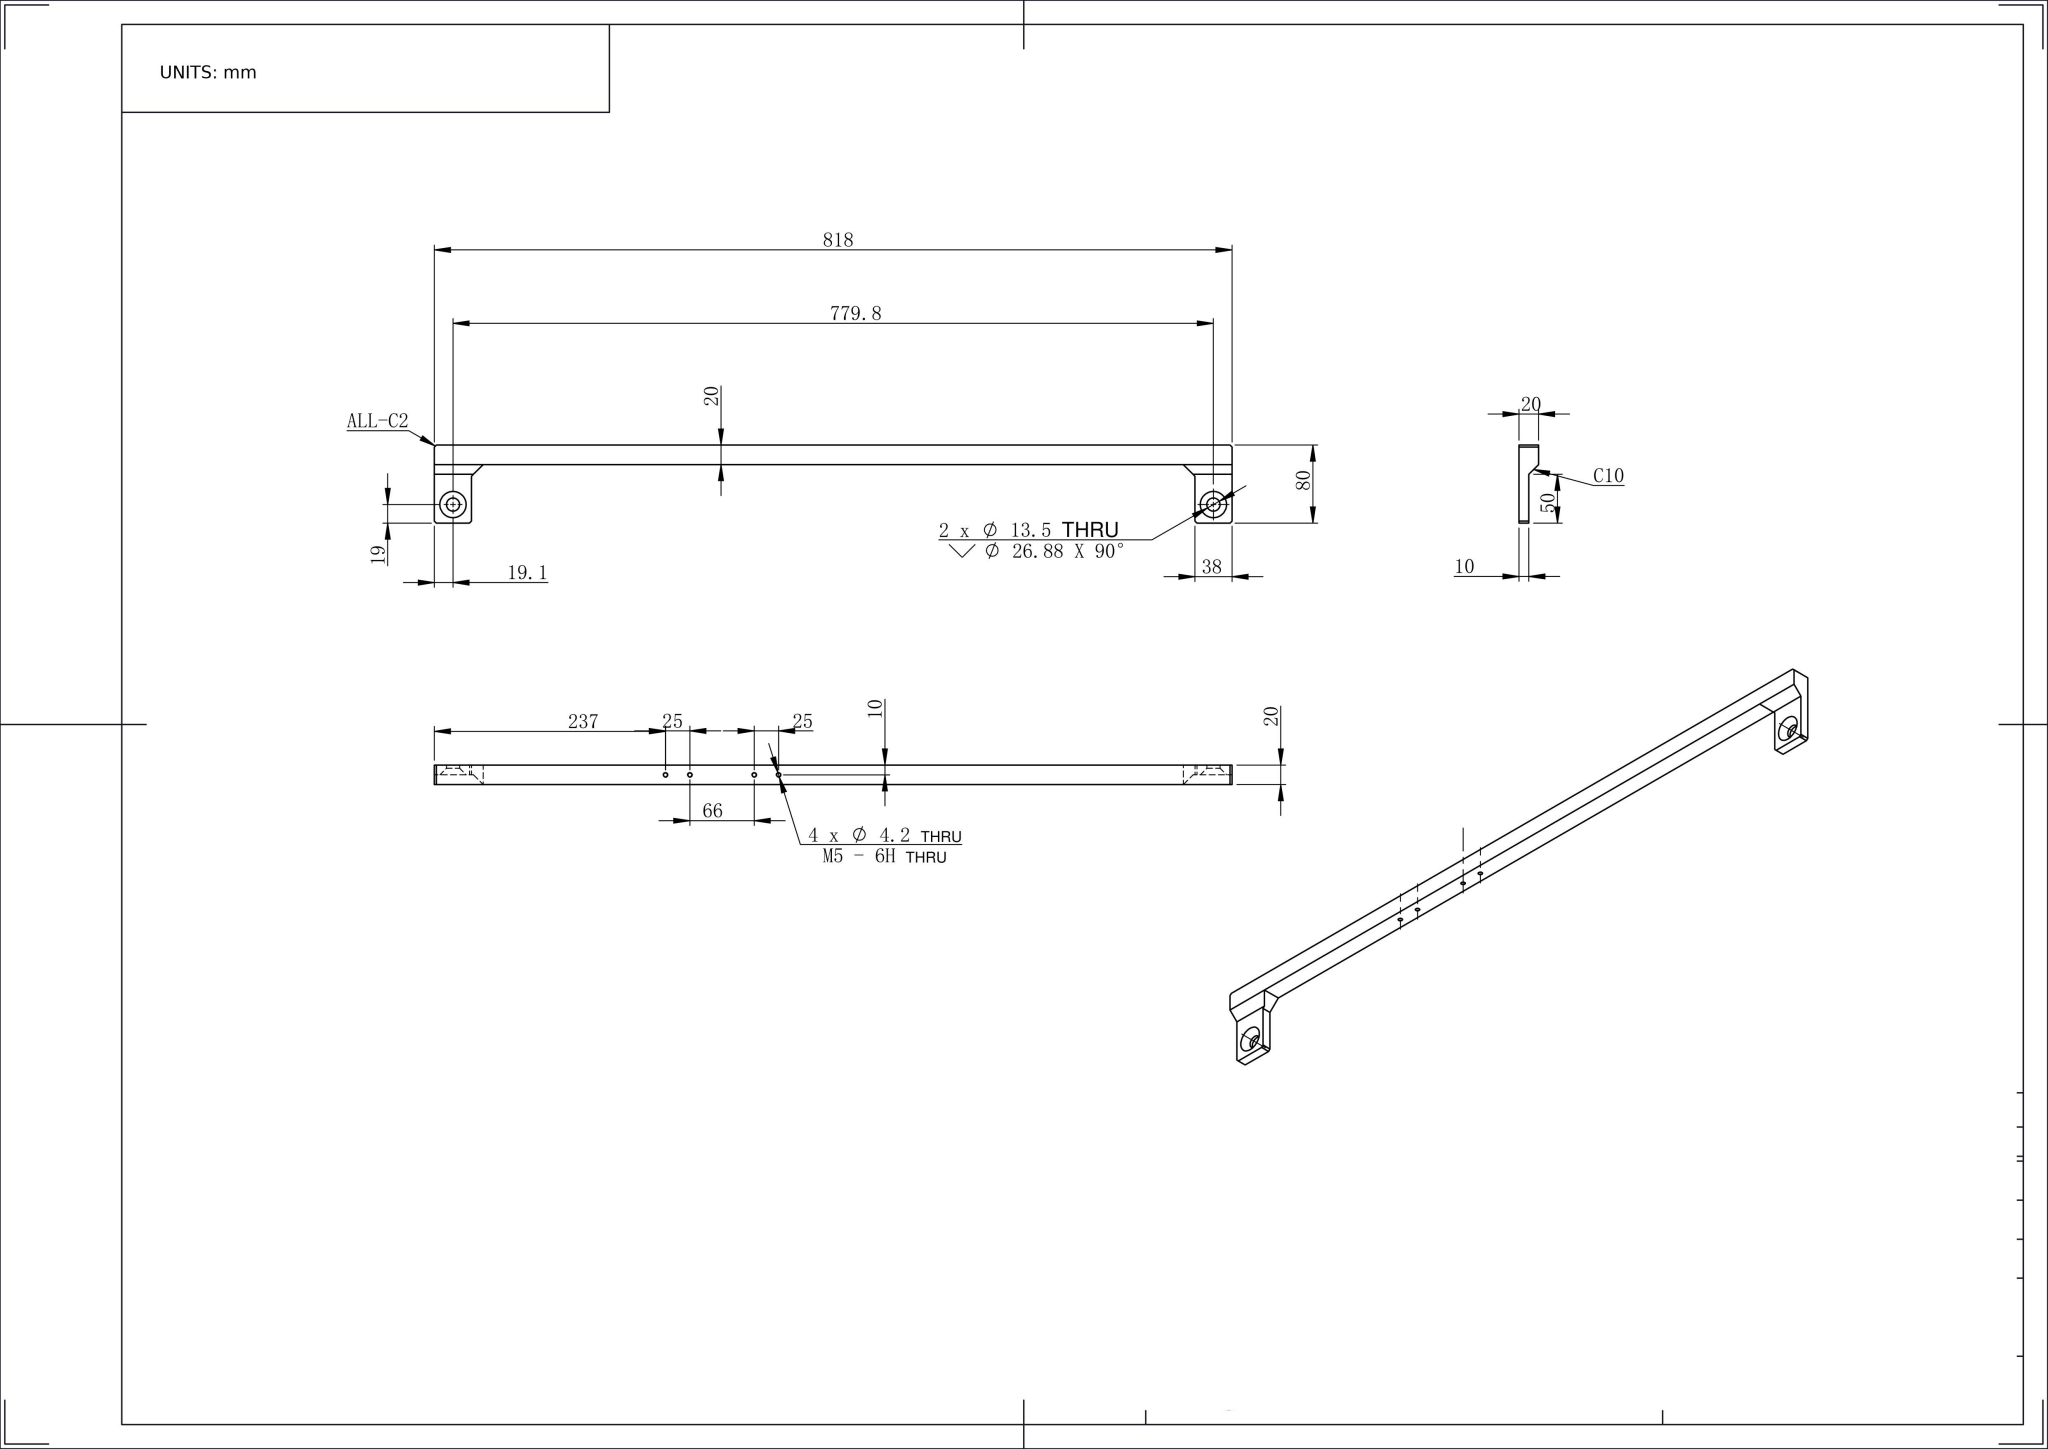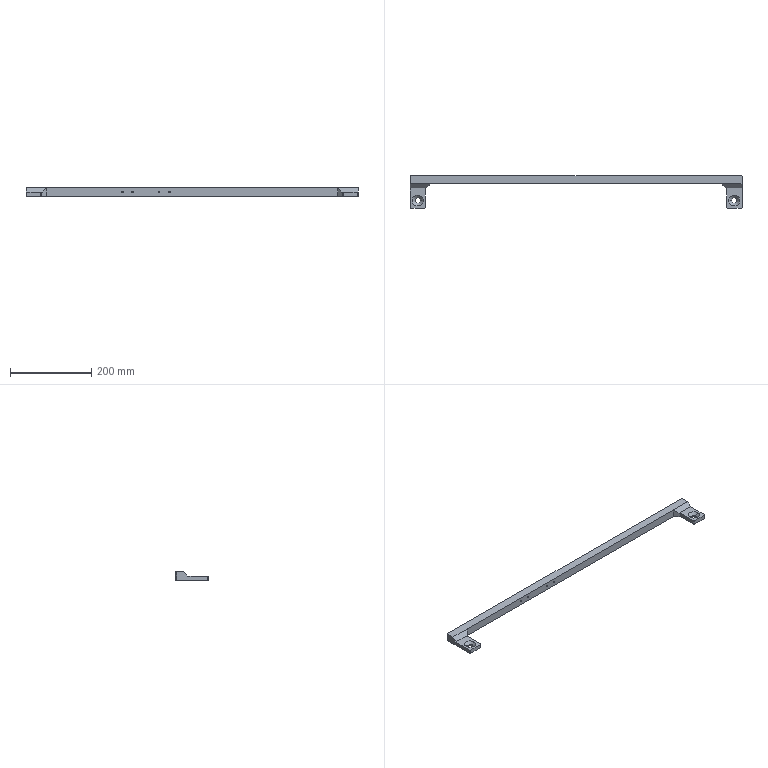Part | NX | mm | 1 solid | 38 faces | box 818 x 80 x 20 mm | volume 372250 mm3 | plane 22 | cylinder 12 | cone 4 | commonest cylinder face diameters 4.2 x8 13.5 x4